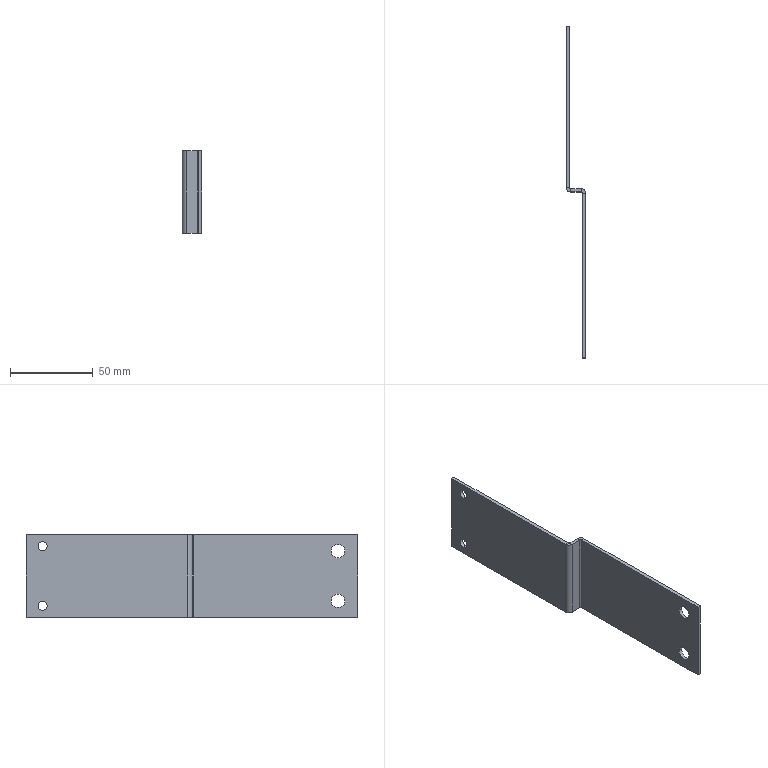Component | SolidWorks | JL001-05-01-010-2 | 1 solid | 30 faces | box 12 x 200 x 50 mm | volume 20545 mm3 | plane 18 | cylinder 12 | commonest cylinder face diameters 8.2 x4 5.5 x4 1.473 x2 5.473 x2
STEP:
#1=COLOUR_RGB('',0.7922,0.8196,0.9333);
#2=FILL_AREA_STYLE_COLOUR('',#1);
#3=FILL_AREA_STYLE('',(#2));
#4=SURFACE_STYLE_FILL_AREA(#3);
#5=SURFACE_SIDE_STYLE('',(#4));
#6=SURFACE_STYLE_USAGE(.BOTH.,#5);
#7=PRESENTATION_STYLE_ASSIGNMENT((#6));
#8=CARTESIAN_POINT('',(1.181,37.319,-0.4724));
#9=VERTEX_POINT('',#8);
#10=CARTESIAN_POINT('',(1.181,37.642,-0.4724));
#11=VERTEX_POINT('',#10);
#12=CARTESIAN_POINT('',(1.181,37.48,-0.4724));
#13=DIRECTION('',(-1.,0.,0.));
#14=DIRECTION('',(0.,1.,0.));
#15=AXIS2_PLACEMENT_3D('',#12,#13,#14);
#16=CIRCLE('',#15,0.1614);
#17=EDGE_CURVE('',#9,#11,#16,.T.);
#18=ORIENTED_EDGE('',*,*,#17,.T.);
#19=CARTESIAN_POINT('',(1.26,37.642,-0.4724));
#20=VERTEX_POINT('',#19);
#21=CARTESIAN_POINT('',(1.26,37.642,-0.4724));
#22=DIRECTION('',(1.,-0.,-0.));
#23=VECTOR('',#22,39.37);
#24=LINE('',#21,#23);
#25=EDGE_CURVE('',#11,#20,#24,.T.);
#26=ORIENTED_EDGE('',*,*,#25,.T.);
#27=CARTESIAN_POINT('',(1.26,37.319,-0.4724));
#28=VERTEX_POINT('',#27);
#29=CARTESIAN_POINT('',(1.26,37.48,-0.4724));
#30=DIRECTION('',(1.,-0.,-0.));
#31=DIRECTION('',(0.,-1.,0.));
#32=AXIS2_PLACEMENT_3D('',#29,#30,#31);
#33=CIRCLE('',#32,0.1614);
#34=EDGE_CURVE('',#20,#28,#33,.T.);
#35=ORIENTED_EDGE('',*,*,#34,.T.);
#36=CARTESIAN_POINT('',(1.26,37.319,-0.4724));
#37=DIRECTION('',(1.,-0.,-0.));
#38=VECTOR('',#37,39.37);
#39=LINE('',#36,#38);
#40=EDGE_CURVE('',#9,#28,#39,.T.);
#41=ORIENTED_EDGE('',*,*,#40,.F.);
#42=EDGE_LOOP('',(#18,#26,#35,#41));
#43=FACE_OUTER_BOUND('',#42,.T.);
#44=CARTESIAN_POINT('',(1.26,37.48,-0.4724));
#45=DIRECTION('',(1.,-0.,-0.));
#46=DIRECTION('',(0.,-1.,0.));
#47=AXIS2_PLACEMENT_3D('',#44,#45,#46);
#48=CYLINDRICAL_SURFACE('',#47,0.1614);
#49=ADVANCED_FACE('',(#43),#48,.F.);
#50=CARTESIAN_POINT('',(1.181,37.319,0.7087));
#51=VERTEX_POINT('',#50);
#52=CARTESIAN_POINT('',(1.181,37.642,0.7087));
#53=VERTEX_POINT('',#52);
#54=CARTESIAN_POINT('',(1.181,37.48,0.7087));
#55=DIRECTION('',(-1.,0.,0.));
#56=DIRECTION('',(0.,1.,0.));
#57=AXIS2_PLACEMENT_3D('',#54,#55,#56);
#58=CIRCLE('',#57,0.1614);
#59=EDGE_CURVE('',#51,#53,#58,.T.);
#60=ORIENTED_EDGE('',*,*,#59,.T.);
#61=CARTESIAN_POINT('',(1.26,37.642,0.7087));
#62=VERTEX_POINT('',#61);
#63=CARTESIAN_POINT('',(1.26,37.642,0.7087));
#64=DIRECTION('',(1.,-0.,-0.));
#65=VECTOR('',#64,39.37);
#66=LINE('',#63,#65);
#67=EDGE_CURVE('',#53,#62,#66,.T.);
#68=ORIENTED_EDGE('',*,*,#67,.T.);
#69=CARTESIAN_POINT('',(1.26,37.319,0.7087));
#70=VERTEX_POINT('',#69);
#71=CARTESIAN_POINT('',(1.26,37.48,0.7087));
#72=DIRECTION('',(1.,-0.,-0.));
#73=DIRECTION('',(0.,-1.,0.));
#74=AXIS2_PLACEMENT_3D('',#71,#72,#73);
#75=CIRCLE('',#74,0.1614);
#76=EDGE_CURVE('',#62,#70,#75,.T.);
#77=ORIENTED_EDGE('',*,*,#76,.T.);
#78=CARTESIAN_POINT('',(1.26,37.319,0.7087));
#79=DIRECTION('',(1.,-0.,-0.));
#80=VECTOR('',#79,39.37);
#81=LINE('',#78,#80);
#82=EDGE_CURVE('',#51,#70,#81,.T.);
#83=ORIENTED_EDGE('',*,*,#82,.F.);
#84=EDGE_LOOP('',(#60,#68,#77,#83));
#85=FACE_OUTER_BOUND('',#84,.T.);
#86=CARTESIAN_POINT('',(1.26,37.48,0.7087));
#87=DIRECTION('',(1.,-0.,-0.));
#88=DIRECTION('',(0.,-1.,0.));
#89=AXIS2_PLACEMENT_3D('',#86,#87,#88);
#90=CYLINDRICAL_SURFACE('',#89,0.1614);
#91=ADVANCED_FACE('',(#85),#90,.F.);
#92=CARTESIAN_POINT('',(0.7874,44.488,-0.6988));
#93=VERTEX_POINT('',#92);
#94=CARTESIAN_POINT('',(0.7874,44.488,-0.4823));
#95=VERTEX_POINT('',#94);
#96=CARTESIAN_POINT('',(0.7874,44.488,-0.5906));
#97=DIRECTION('',(1.,0.,-0.));
#98=DIRECTION('',(0.,0.,1.));
#99=AXIS2_PLACEMENT_3D('',#96,#97,#98);
#100=CIRCLE('',#99,0.1083);
#101=EDGE_CURVE('',#93,#95,#100,.T.);
#102=ORIENTED_EDGE('',*,*,#101,.F.);
#103=CARTESIAN_POINT('',(0.8661,44.488,-0.6988));
#104=VERTEX_POINT('',#103);
#105=CARTESIAN_POINT('',(0.8661,44.488,-0.6988));
#106=DIRECTION('',(1.,0.,-0.));
#107=VECTOR('',#106,39.37);
#108=LINE('',#105,#107);
#109=EDGE_CURVE('',#93,#104,#108,.T.);
#110=ORIENTED_EDGE('',*,*,#109,.T.);
#111=CARTESIAN_POINT('',(0.8661,44.488,-0.4823));
#112=VERTEX_POINT('',#111);
#113=CARTESIAN_POINT('',(0.8661,44.488,-0.5906));
#114=DIRECTION('',(1.,0.,-0.));
#115=DIRECTION('',(0.,0.,1.));
#116=AXIS2_PLACEMENT_3D('',#113,#114,#115);
#117=CIRCLE('',#116,0.1083);
#118=EDGE_CURVE('',#104,#112,#117,.T.);
#119=ORIENTED_EDGE('',*,*,#118,.T.);
#120=CARTESIAN_POINT('',(0.8661,44.488,-0.4823));
#121=DIRECTION('',(1.,0.,-0.));
#122=VECTOR('',#121,39.37);
#123=LINE('',#120,#122);
#124=EDGE_CURVE('',#95,#112,#123,.T.);
#125=ORIENTED_EDGE('',*,*,#124,.F.);
#126=EDGE_LOOP('',(#102,#110,#119,#125));
#127=FACE_OUTER_BOUND('',#126,.T.);
#128=CARTESIAN_POINT('',(0.8661,44.488,-0.5906));
#129=DIRECTION('',(1.,0.,-0.));
#130=DIRECTION('',(0.,0.,1.));
#131=AXIS2_PLACEMENT_3D('',#128,#129,#130);
#132=CYLINDRICAL_SURFACE('',#131,0.1083);
#133=ADVANCED_FACE('',(#127),#132,.F.);
#134=CARTESIAN_POINT('',(0.7874,44.488,0.7185));
#135=VERTEX_POINT('',#134);
#136=CARTESIAN_POINT('',(0.7874,44.488,0.935));
#137=VERTEX_POINT('',#136);
#138=CARTESIAN_POINT('',(0.7874,44.488,0.8268));
#139=DIRECTION('',(1.,0.,-0.));
#140=DIRECTION('',(0.,0.,1.));
#141=AXIS2_PLACEMENT_3D('',#138,#139,#140);
#142=CIRCLE('',#141,0.1083);
#143=EDGE_CURVE('',#135,#137,#142,.T.);
#144=ORIENTED_EDGE('',*,*,#143,.F.);
#145=CARTESIAN_POINT('',(0.8661,44.488,0.7185));
#146=VERTEX_POINT('',#145);
#147=CARTESIAN_POINT('',(0.8661,44.488,0.7185));
#148=DIRECTION('',(1.,0.,-0.));
#149=VECTOR('',#148,39.37);
#150=LINE('',#147,#149);
#151=EDGE_CURVE('',#135,#146,#150,.T.);
#152=ORIENTED_EDGE('',*,*,#151,.T.);
#153=CARTESIAN_POINT('',(0.8661,44.488,0.935));
#154=VERTEX_POINT('',#153);
#155=CARTESIAN_POINT('',(0.8661,44.488,0.8268));
#156=DIRECTION('',(1.,0.,-0.));
#157=DIRECTION('',(0.,0.,1.));
#158=AXIS2_PLACEMENT_3D('',#155,#156,#157);
#159=CIRCLE('',#158,0.1083);
#160=EDGE_CURVE('',#146,#154,#159,.T.);
#161=ORIENTED_EDGE('',*,*,#160,.T.);
#162=CARTESIAN_POINT('',(0.8661,44.488,0.935));
#163=DIRECTION('',(1.,0.,-0.));
#164=VECTOR('',#163,39.37);
#165=LINE('',#162,#164);
#166=EDGE_CURVE('',#137,#154,#165,.T.);
#167=ORIENTED_EDGE('',*,*,#166,.F.);
#168=EDGE_LOOP('',(#144,#152,#161,#167));
#169=FACE_OUTER_BOUND('',#168,.T.);
#170=CARTESIAN_POINT('',(0.8661,44.488,0.8268));
#171=DIRECTION('',(1.,0.,-0.));
#172=DIRECTION('',(0.,0.,1.));
#173=AXIS2_PLACEMENT_3D('',#170,#171,#172);
#174=CYLINDRICAL_SURFACE('',#173,0.1083);
#175=ADVANCED_FACE('',(#169),#174,.F.);
#176=CARTESIAN_POINT('',(0.8951,40.945,-0.8661));
#177=VERTEX_POINT('',#176);
#178=CARTESIAN_POINT('',(0.8951,41.024,-0.8661));
#179=VERTEX_POINT('',#178);
#180=CARTESIAN_POINT('',(0.8951,40.945,-0.8661));
#181=DIRECTION('',(0.,1.,0.));
#182=VECTOR('',#181,39.37);
#183=LINE('',#180,#182);
#184=EDGE_CURVE('',#177,#179,#183,.T.);
#185=ORIENTED_EDGE('',*,*,#184,.F.);
#186=CARTESIAN_POINT('',(0.7874,41.053,-0.8661));
#187=VERTEX_POINT('',#186);
#188=CARTESIAN_POINT('',(0.8951,41.053,-0.8661));
#189=DIRECTION('',(0.,0.,1.));
#190=DIRECTION('',(1.,0.,0.));
#191=AXIS2_PLACEMENT_3D('',#188,#189,#190);
#192=CIRCLE('',#191,0.1077);
#193=EDGE_CURVE('',#187,#177,#192,.T.);
#194=ORIENTED_EDGE('',*,*,#193,.F.);
#195=CARTESIAN_POINT('',(0.8661,41.053,-0.8661));
#196=VERTEX_POINT('',#195);
#197=CARTESIAN_POINT('',(0.8661,41.053,-0.8661));
#198=DIRECTION('',(-1.,0.,0.));
#199=VECTOR('',#198,39.37);
#200=LINE('',#197,#199);
#201=EDGE_CURVE('',#196,#187,#200,.T.);
#202=ORIENTED_EDGE('',*,*,#201,.F.);
#203=CARTESIAN_POINT('',(0.8951,41.053,-0.8661));
#204=DIRECTION('',(0.,0.,1.));
#205=DIRECTION('',(1.,0.,0.));
#206=AXIS2_PLACEMENT_3D('',#203,#204,#205);
#207=CIRCLE('',#206,0.029);
#208=EDGE_CURVE('',#196,#179,#207,.T.);
#209=ORIENTED_EDGE('',*,*,#208,.T.);
#210=EDGE_LOOP('',(#185,#194,#202,#209));
#211=FACE_OUTER_BOUND('',#210,.T.);
#212=CARTESIAN_POINT('',(0.8951,40.945,-0.8661));
#213=DIRECTION('',(-0.,0.,-1.));
#214=DIRECTION('',(1.,0.,-0.));
#215=AXIS2_PLACEMENT_3D('',#212,#213,#214);
#216=PLANE('',#215);
#217=ADVANCED_FACE('',(#211),#216,.T.);
#218=CARTESIAN_POINT('',(1.152,40.945,-0.8661));
#219=VERTEX_POINT('',#218);
#220=CARTESIAN_POINT('',(0.7874,40.945,-0.8661));
#221=DIRECTION('',(1.,0.,-0.));
#222=VECTOR('',#221,39.37);
#223=LINE('',#220,#222);
#224=EDGE_CURVE('',#177,#219,#223,.T.);
#225=ORIENTED_EDGE('',*,*,#224,.F.);
#226=ORIENTED_EDGE('',*,*,#184,.T.);
#227=CARTESIAN_POINT('',(1.152,41.024,-0.8661));
#228=VERTEX_POINT('',#227);
#229=CARTESIAN_POINT('',(0.7874,41.024,-0.8661));
#230=DIRECTION('',(1.,0.,-0.));
#231=VECTOR('',#230,39.37);
#232=LINE('',#229,#231);
#233=EDGE_CURVE('',#179,#228,#232,.T.);
#234=ORIENTED_EDGE('',*,*,#233,.T.);
#235=CARTESIAN_POINT('',(1.152,41.024,-0.8661));
#236=DIRECTION('',(0.,-1.,0.));
#237=VECTOR('',#236,39.37);
#238=LINE('',#235,#237);
#239=EDGE_CURVE('',#228,#219,#238,.T.);
#240=ORIENTED_EDGE('',*,*,#239,.T.);
#241=EDGE_LOOP('',(#225,#226,#234,#240));
#242=FACE_OUTER_BOUND('',#241,.T.);
#243=CARTESIAN_POINT('',(0.8661,41.053,-0.8661));
#244=DIRECTION('',(-0.,0.,-1.));
#245=DIRECTION('',(1.,0.,-0.));
#246=AXIS2_PLACEMENT_3D('',#243,#244,#245);
#247=PLANE('',#246);
#248=ADVANCED_FACE('',(#242),#247,.T.);
#249=CARTESIAN_POINT('',(0.7874,41.053,1.102));
#250=VERTEX_POINT('',#249);
#251=CARTESIAN_POINT('',(0.8661,41.053,1.102));
#252=VERTEX_POINT('',#251);
#253=CARTESIAN_POINT('',(0.7874,41.053,1.102));
#254=DIRECTION('',(1.,0.,-0.));
#255=VECTOR('',#254,39.37);
#256=LINE('',#253,#255);
#257=EDGE_CURVE('',#250,#252,#256,.T.);
#258=ORIENTED_EDGE('',*,*,#257,.F.);
#259=CARTESIAN_POINT('',(0.8951,40.945,1.102));
#260=VERTEX_POINT('',#259);
#261=CARTESIAN_POINT('',(0.8951,41.053,1.102));
#262=DIRECTION('',(0.,0.,1.));
#263=DIRECTION('',(1.,0.,0.));
#264=AXIS2_PLACEMENT_3D('',#261,#262,#263);
#265=CIRCLE('',#264,0.1077);
#266=EDGE_CURVE('',#250,#260,#265,.T.);
#267=ORIENTED_EDGE('',*,*,#266,.T.);
#268=CARTESIAN_POINT('',(0.8951,41.024,1.102));
#269=VERTEX_POINT('',#268);
#270=CARTESIAN_POINT('',(0.8951,41.024,1.102));
#271=DIRECTION('',(0.,-1.,0.));
#272=VECTOR('',#271,39.37);
#273=LINE('',#270,#272);
#274=EDGE_CURVE('',#269,#260,#273,.T.);
#275=ORIENTED_EDGE('',*,*,#274,.F.);
#276=CARTESIAN_POINT('',(0.8951,41.053,1.102));
#277=DIRECTION('',(0.,0.,1.));
#278=DIRECTION('',(1.,0.,0.));
#279=AXIS2_PLACEMENT_3D('',#276,#277,#278);
#280=CIRCLE('',#279,0.029);
#281=EDGE_CURVE('',#252,#269,#280,.T.);
#282=ORIENTED_EDGE('',*,*,#281,.F.);
#283=EDGE_LOOP('',(#258,#267,#275,#282));
#284=FACE_OUTER_BOUND('',#283,.T.);
#285=CARTESIAN_POINT('',(0.7874,41.053,1.102));
#286=DIRECTION('',(0.,0.,1.));
#287=DIRECTION('',(-1.,0.,0.));
#288=AXIS2_PLACEMENT_3D('',#285,#286,#287);
#289=PLANE('',#288);
#290=ADVANCED_FACE('',(#284),#289,.T.);
#291=CARTESIAN_POINT('',(0.7874,44.882,1.102));
#292=VERTEX_POINT('',#291);
#293=CARTESIAN_POINT('',(0.7874,44.882,1.102));
#294=DIRECTION('',(0.,-1.,0.));
#295=VECTOR('',#294,39.37);
#296=LINE('',#293,#295);
#297=EDGE_CURVE('',#292,#250,#296,.T.);
#298=ORIENTED_EDGE('',*,*,#297,.T.);
#299=ORIENTED_EDGE('',*,*,#257,.T.);
#300=CARTESIAN_POINT('',(0.8661,44.882,1.102));
#301=VERTEX_POINT('',#300);
#302=CARTESIAN_POINT('',(0.8661,44.882,1.102));
#303=DIRECTION('',(0.,-1.,0.));
#304=VECTOR('',#303,39.37);
#305=LINE('',#302,#304);
#306=EDGE_CURVE('',#301,#252,#305,.T.);
#307=ORIENTED_EDGE('',*,*,#306,.F.);
#308=CARTESIAN_POINT('',(0.8661,44.882,1.102));
#309=DIRECTION('',(-1.,0.,0.));
#310=VECTOR('',#309,39.37);
#311=LINE('',#308,#310);
#312=EDGE_CURVE('',#301,#292,#311,.T.);
#313=ORIENTED_EDGE('',*,*,#312,.T.);
#314=EDGE_LOOP('',(#298,#299,#307,#313));
#315=FACE_OUTER_BOUND('',#314,.T.);
#316=CARTESIAN_POINT('',(0.8951,41.024,1.102));
#317=DIRECTION('',(0.,0.,1.));
#318=DIRECTION('',(-1.,0.,0.));
#319=AXIS2_PLACEMENT_3D('',#316,#317,#318);
#320=PLANE('',#319);
#321=ADVANCED_FACE('',(#315),#320,.T.);
#322=CARTESIAN_POINT('',(1.181,40.916,-0.8661));
#323=VERTEX_POINT('',#322);
#324=CARTESIAN_POINT('',(1.26,40.916,-0.8661));
#325=VERTEX_POINT('',#324);
#326=CARTESIAN_POINT('',(1.181,40.916,-0.8661));
#327=DIRECTION('',(1.,0.,-0.));
#328=VECTOR('',#327,39.37);
#329=LINE('',#326,#328);
#330=EDGE_CURVE('',#323,#325,#329,.T.);
#331=ORIENTED_EDGE('',*,*,#330,.F.);
#332=CARTESIAN_POINT('',(1.152,40.916,-0.8661));
#333=DIRECTION('',(-0.,0.,-1.));
#334=DIRECTION('',(-1.,0.,0.));
#335=AXIS2_PLACEMENT_3D('',#332,#333,#334);
#336=CIRCLE('',#335,0.029);
#337=EDGE_CURVE('',#219,#323,#336,.T.);
#338=ORIENTED_EDGE('',*,*,#337,.F.);
#339=ORIENTED_EDGE('',*,*,#239,.F.);
#340=CARTESIAN_POINT('',(1.152,40.916,-0.8661));
#341=DIRECTION('',(-0.,0.,-1.));
#342=DIRECTION('',(1.,0.,0.));
#343=AXIS2_PLACEMENT_3D('',#340,#341,#342);
#344=CIRCLE('',#343,0.1077);
#345=EDGE_CURVE('',#228,#325,#344,.T.);
#346=ORIENTED_EDGE('',*,*,#345,.T.);
#347=EDGE_LOOP('',(#331,#338,#339,#346));
#348=FACE_OUTER_BOUND('',#347,.T.);
#349=CARTESIAN_POINT('',(1.181,40.916,-0.8661));
#350=DIRECTION('',(-0.,0.,-1.));
#351=DIRECTION('',(1.,0.,-0.));
#352=AXIS2_PLACEMENT_3D('',#349,#350,#351);
#353=PLANE('',#352);
#354=ADVANCED_FACE('',(#348),#353,.T.);
#355=CARTESIAN_POINT('',(1.181,37.008,-0.8661));
#356=VERTEX_POINT('',#355);
#357=CARTESIAN_POINT('',(1.181,40.945,-0.8661));
#358=DIRECTION('',(-0.,-1.,0.));
#359=VECTOR('',#358,39.37);
#360=LINE('',#357,#359);
#361=EDGE_CURVE('',#323,#356,#360,.T.);
#362=ORIENTED_EDGE('',*,*,#361,.F.);
#363=ORIENTED_EDGE('',*,*,#330,.T.);
#364=CARTESIAN_POINT('',(1.26,37.008,-0.8661));
#365=VERTEX_POINT('',#364);
#366=CARTESIAN_POINT('',(1.26,40.945,-0.8661));
#367=DIRECTION('',(-0.,-1.,0.));
#368=VECTOR('',#367,39.37);
#369=LINE('',#366,#368);
#370=EDGE_CURVE('',#325,#365,#369,.T.);
#371=ORIENTED_EDGE('',*,*,#370,.T.);
#372=CARTESIAN_POINT('',(1.181,37.008,-0.8661));
#373=DIRECTION('',(1.,0.,-0.));
#374=VECTOR('',#373,39.37);
#375=LINE('',#372,#374);
#376=EDGE_CURVE('',#356,#365,#375,.T.);
#377=ORIENTED_EDGE('',*,*,#376,.F.);
#378=EDGE_LOOP('',(#362,#363,#371,#377));
#379=FACE_OUTER_BOUND('',#378,.T.);
#380=CARTESIAN_POINT('',(1.152,41.024,-0.8661));
#381=DIRECTION('',(-0.,0.,-1.));
#382=DIRECTION('',(1.,0.,-0.));
#383=AXIS2_PLACEMENT_3D('',#380,#381,#382);
#384=PLANE('',#383);
#385=ADVANCED_FACE('',(#379),#384,.T.);
#386=CARTESIAN_POINT('',(1.152,40.945,1.102));
#387=VERTEX_POINT('',#386);
#388=CARTESIAN_POINT('',(1.152,41.024,1.102));
#389=VERTEX_POINT('',#388);
#390=CARTESIAN_POINT('',(1.152,40.945,1.102));
#391=DIRECTION('',(0.,1.,0.));
#392=VECTOR('',#391,39.37);
#393=LINE('',#390,#392);
#394=EDGE_CURVE('',#387,#389,#393,.T.);
#395=ORIENTED_EDGE('',*,*,#394,.F.);
#396=CARTESIAN_POINT('',(1.181,40.916,1.102));
#397=VERTEX_POINT('',#396);
#398=CARTESIAN_POINT('',(1.152,40.916,1.102));
#399=DIRECTION('',(-0.,0.,-1.));
#400=DIRECTION('',(-1.,0.,0.));
#401=AXIS2_PLACEMENT_3D('',#398,#399,#400);
#402=CIRCLE('',#401,0.029);
#403=EDGE_CURVE('',#387,#397,#402,.T.);
#404=ORIENTED_EDGE('',*,*,#403,.T.);
#405=CARTESIAN_POINT('',(1.26,40.916,1.102));
#406=VERTEX_POINT('',#405);
#407=CARTESIAN_POINT('',(1.26,40.916,1.102));
#408=DIRECTION('',(-1.,0.,0.));
#409=VECTOR('',#408,39.37);
#410=LINE('',#407,#409);
#411=EDGE_CURVE('',#406,#397,#410,.T.);
#412=ORIENTED_EDGE('',*,*,#411,.F.);
#413=CARTESIAN_POINT('',(1.152,40.916,1.102));
#414=DIRECTION('',(-0.,0.,-1.));
#415=DIRECTION('',(1.,0.,0.));
#416=AXIS2_PLACEMENT_3D('',#413,#414,#415);
#417=CIRCLE('',#416,0.1077);
#418=EDGE_CURVE('',#389,#406,#417,.T.);
#419=ORIENTED_EDGE('',*,*,#418,.F.);
#420=EDGE_LOOP('',(#395,#404,#412,#419));
#421=FACE_OUTER_BOUND('',#420,.T.);
#422=CARTESIAN_POINT('',(1.152,40.945,1.102));
#423=DIRECTION('',(0.,0.,1.));
#424=DIRECTION('',(-1.,0.,0.));
#425=AXIS2_PLACEMENT_3D('',#422,#423,#424);
#426=PLANE('',#425);
#427=ADVANCED_FACE('',(#421),#426,.T.);
#428=CARTESIAN_POINT('',(0.7874,40.945,1.102));
#429=DIRECTION('',(1.,0.,-0.));
#430=VECTOR('',#429,39.37);
#431=LINE('',#428,#430);
#432=EDGE_CURVE('',#260,#387,#431,.T.);
#433=ORIENTED_EDGE('',*,*,#432,.T.);
#434=ORIENTED_EDGE('',*,*,#394,.T.);
#435=CARTESIAN_POINT('',(0.7874,41.024,1.102));
#436=DIRECTION('',(1.,0.,-0.));
#437=VECTOR('',#436,39.37);
#438=LINE('',#435,#437);
#439=EDGE_CURVE('',#269,#389,#438,.T.);
#440=ORIENTED_EDGE('',*,*,#439,.F.);
#441=ORIENTED_EDGE('',*,*,#274,.T.);
#442=EDGE_LOOP('',(#433,#434,#440,#441));
#443=FACE_OUTER_BOUND('',#442,.T.);
#444=CARTESIAN_POINT('',(1.26,40.916,1.102));
#445=DIRECTION('',(0.,0.,1.));
#446=DIRECTION('',(-1.,0.,0.));
#447=AXIS2_PLACEMENT_3D('',#444,#445,#446);
#448=PLANE('',#447);
#449=ADVANCED_FACE('',(#443),#448,.T.);
#450=CARTESIAN_POINT('',(1.26,37.48,-0.4724));
#451=DIRECTION('',(1.,-0.,-0.));
#452=DIRECTION('',(0.,-1.,0.));
#453=AXIS2_PLACEMENT_3D('',#450,#451,#452);
#454=CIRCLE('',#453,0.1614);
#455=EDGE_CURVE('',#28,#20,#454,.T.);
#456=ORIENTED_EDGE('',*,*,#455,.F.);
#457=ORIENTED_EDGE('',*,*,#34,.F.);
#458=EDGE_LOOP('',(#456,#457));
#459=FACE_BOUND('',#458,.T.);
#460=CARTESIAN_POINT('',(1.26,37.48,0.7087));
#461=DIRECTION('',(1.,-0.,-0.));
#462=DIRECTION('',(0.,-1.,0.));
#463=AXIS2_PLACEMENT_3D('',#460,#461,#462);
#464=CIRCLE('',#463,0.1614);
#465=EDGE_CURVE('',#70,#62,#464,.T.);
#466=ORIENTED_EDGE('',*,*,#465,.F.);
#467=ORIENTED_EDGE('',*,*,#76,.F.);
#468=EDGE_LOOP('',(#466,#467));
#469=FACE_BOUND('',#468,.T.);
#470=CARTESIAN_POINT('',(1.26,37.008,1.102));
#471=VERTEX_POINT('',#470);
#472=CARTESIAN_POINT('',(1.26,40.945,1.102));
#473=DIRECTION('',(-0.,-1.,0.));
#474=VECTOR('',#473,39.37);
#475=LINE('',#472,#474);
#476=EDGE_CURVE('',#406,#471,#475,.T.);
#477=ORIENTED_EDGE('',*,*,#476,.T.);
#478=CARTESIAN_POINT('',(1.26,37.008,-0.8661));
#479=DIRECTION('',(0.,0.,1.));
#480=VECTOR('',#479,39.37);
#481=LINE('',#478,#480);
#482=EDGE_CURVE('',#365,#471,#481,.T.);
#483=ORIENTED_EDGE('',*,*,#482,.F.);
#484=ORIENTED_EDGE('',*,*,#370,.F.);
#485=CARTESIAN_POINT('',(1.26,40.916,-0.8661));
#486=DIRECTION('',(0.,0.,1.));
#487=VECTOR('',#486,39.37);
#488=LINE('',#485,#487);
#489=EDGE_CURVE('',#325,#406,#488,.T.);
#490=ORIENTED_EDGE('',*,*,#489,.T.);
#491=EDGE_LOOP('',(#477,#483,#484,#490));
#492=FACE_OUTER_BOUND('',#491,.T.);
#493=CARTESIAN_POINT('',(1.26,40.945,-0.8661));
#494=DIRECTION('',(-1.,0.,0.));
#495=DIRECTION('',(0.,1.,-0.));
#496=AXIS2_PLACEMENT_3D('',#493,#494,#495);
#497=PLANE('',#496);
#498=ADVANCED_FACE('',(#459,#469,#492),#497,.F.);
#499=CARTESIAN_POINT('',(1.181,37.008,1.102));
#500=VERTEX_POINT('',#499);
#501=CARTESIAN_POINT('',(1.181,37.008,1.102));
#502=DIRECTION('',(1.,0.,-0.));
#503=VECTOR('',#502,39.37);
#504=LINE('',#501,#503);
#505=EDGE_CURVE('',#500,#471,#504,.T.);
#506=ORIENTED_EDGE('',*,*,#505,.F.);
#507=CARTESIAN_POINT('',(1.181,37.008,-0.8661));
#508=DIRECTION('',(0.,0.,1.));
#509=VECTOR('',#508,39.37);
#510=LINE('',#507,#509);
#511=EDGE_CURVE('',#356,#500,#510,.T.);
#512=ORIENTED_EDGE('',*,*,#511,.F.);
#513=ORIENTED_EDGE('',*,*,#376,.T.);
#514=ORIENTED_EDGE('',*,*,#482,.T.);
#515=EDGE_LOOP('',(#506,#512,#513,#514));
#516=FACE_OUTER_BOUND('',#515,.T.);
#517=CARTESIAN_POINT('',(1.181,37.008,-0.8661));
#518=DIRECTION('',(0.,-1.,0.));
#519=DIRECTION('',(-1.,0.,0.));
#520=AXIS2_PLACEMENT_3D('',#517,#518,#519);
#521=PLANE('',#520);
#522=ADVANCED_FACE('',(#516),#521,.T.);
#523=ORIENTED_EDGE('',*,*,#17,.F.);
#524=CARTESIAN_POINT('',(1.181,37.48,-0.4724));
#525=DIRECTION('',(-1.,0.,0.));
#526=DIRECTION('',(0.,1.,0.));
#527=AXIS2_PLACEMENT_3D('',#524,#525,#526);
#528=CIRCLE('',#527,0.1614);
#529=EDGE_CURVE('',#11,#9,#528,.T.);
#530=ORIENTED_EDGE('',*,*,#529,.F.);
#531=EDGE_LOOP('',(#523,#530));
#532=FACE_BOUND('',#531,.T.);
#533=ORIENTED_EDGE('',*,*,#59,.F.);
#534=CARTESIAN_POINT('',(1.181,37.48,0.7087));
#535=DIRECTION('',(-1.,0.,0.));
#536=DIRECTION('',(0.,1.,0.));
#537=AXIS2_PLACEMENT_3D('',#534,#535,#536);
#538=CIRCLE('',#537,0.1614);
#539=EDGE_CURVE('',#53,#51,#538,.T.);
#540=ORIENTED_EDGE('',*,*,#539,.F.);
#541=EDGE_LOOP('',(#533,#540));
#542=FACE_BOUND('',#541,.T.);
#543=CARTESIAN_POINT('',(1.181,40.945,1.102));
#544=DIRECTION('',(-0.,-1.,0.));
#545=VECTOR('',#544,39.37);
#546=LINE('',#543,#545);
#547=EDGE_CURVE('',#397,#500,#546,.T.);
#548=ORIENTED_EDGE('',*,*,#547,.F.);
#549=CARTESIAN_POINT('',(1.181,40.916,-0.8661));
#550=DIRECTION('',(0.,0.,1.));
#551=VECTOR('',#550,39.37);
#552=LINE('',#549,#551);
#553=EDGE_CURVE('',#323,#397,#552,.T.);
#554=ORIENTED_EDGE('',*,*,#553,.F.);
#555=ORIENTED_EDGE('',*,*,#361,.T.);
#556=ORIENTED_EDGE('',*,*,#511,.T.);
#557=EDGE_LOOP('',(#548,#554,#555,#556));
#558=FACE_OUTER_BOUND('',#557,.T.);
#559=CARTESIAN_POINT('',(1.181,40.945,-0.8661));
#560=DIRECTION('',(-1.,0.,0.));
#561=DIRECTION('',(0.,1.,-0.));
#562=AXIS2_PLACEMENT_3D('',#559,#560,#561);
#563=PLANE('',#562);
#564=ADVANCED_FACE('',(#532,#542,#558),#563,.T.);
#565=ORIENTED_EDGE('',*,*,#403,.F.);
#566=CARTESIAN_POINT('',(1.152,40.945,-0.8661));
#567=DIRECTION('',(0.,0.,1.));
#568=VECTOR('',#567,39.37);
#569=LINE('',#566,#568);
#570=EDGE_CURVE('',#219,#387,#569,.T.);
#571=ORIENTED_EDGE('',*,*,#570,.F.);
#572=ORIENTED_EDGE('',*,*,#337,.T.);
#573=ORIENTED_EDGE('',*,*,#553,.T.);
#574=EDGE_LOOP('',(#565,#571,#572,#573));
#575=FACE_OUTER_BOUND('',#574,.T.);
#576=CARTESIAN_POINT('',(1.152,40.916,-0.8661));
#577=DIRECTION('',(0.,0.,1.));
#578=DIRECTION('',(-1.,0.,0.));
#579=AXIS2_PLACEMENT_3D('',#576,#577,#578);
#580=CYLINDRICAL_SURFACE('',#579,0.029);
#581=ADVANCED_FACE('',(#575),#580,.F.);
#582=ORIENTED_EDGE('',*,*,#432,.F.);
#583=CARTESIAN_POINT('',(0.8951,40.945,-0.8661));
#584=DIRECTION('',(0.,0.,1.));
#585=VECTOR('',#584,39.37);
#586=LINE('',#583,#585);
#587=EDGE_CURVE('',#177,#260,#586,.T.);
#588=ORIENTED_EDGE('',*,*,#587,.F.);
#589=ORIENTED_EDGE('',*,*,#224,.T.);
#590=ORIENTED_EDGE('',*,*,#570,.T.);
#591=EDGE_LOOP('',(#582,#588,#589,#590));
#592=FACE_OUTER_BOUND('',#591,.T.);
#593=CARTESIAN_POINT('',(0.7874,40.945,-0.8661));
#594=DIRECTION('',(0.,-1.,0.));
#595=DIRECTION('',(-1.,0.,0.));
#596=AXIS2_PLACEMENT_3D('',#593,#594,#595);
#597=PLANE('',#596);
#598=ADVANCED_FACE('',(#592),#597,.T.);
#599=ORIENTED_EDGE('',*,*,#266,.F.);
#600=CARTESIAN_POINT('',(0.7874,41.053,-0.8661));
#601=DIRECTION('',(0.,0.,1.));
#602=VECTOR('',#601,39.37);
#603=LINE('',#600,#602);
#604=EDGE_CURVE('',#187,#250,#603,.T.);
#605=ORIENTED_EDGE('',*,*,#604,.F.);
#606=ORIENTED_EDGE('',*,*,#193,.T.);
#607=ORIENTED_EDGE('',*,*,#587,.T.);
#608=EDGE_LOOP('',(#599,#605,#606,#607));
#609=FACE_OUTER_BOUND('',#608,.T.);
#610=CARTESIAN_POINT('',(0.8951,41.053,-0.8661));
#611=DIRECTION('',(0.,0.,1.));
#612=DIRECTION('',(-1.,0.,0.));
#613=AXIS2_PLACEMENT_3D('',#610,#611,#612);
#614=CYLINDRICAL_SURFACE('',#613,0.1077);
#615=ADVANCED_FACE('',(#609),#614,.T.);
#616=CARTESIAN_POINT('',(0.7874,44.488,-0.5906));
#617=DIRECTION('',(1.,0.,-0.));
#618=DIRECTION('',(0.,0.,1.));
#619=AXIS2_PLACEMENT_3D('',#616,#617,#618);
#620=CIRCLE('',#619,0.1083);
#621=EDGE_CURVE('',#95,#93,#620,.T.);
#622=ORIENTED_EDGE('',*,*,#621,.T.);
#623=ORIENTED_EDGE('',*,*,#101,.T.);
#624=EDGE_LOOP('',(#622,#623));
#625=FACE_BOUND('',#624,.T.);
#626=CARTESIAN_POINT('',(0.7874,44.488,0.8268));
#627=DIRECTION('',(1.,0.,-0.));
#628=DIRECTION('',(0.,0.,1.));
#629=AXIS2_PLACEMENT_3D('',#626,#627,#628);
#630=CIRCLE('',#629,0.1083);
#631=EDGE_CURVE('',#137,#135,#630,.T.);
#632=ORIENTED_EDGE('',*,*,#631,.T.);
#633=ORIENTED_EDGE('',*,*,#143,.T.);
#634=EDGE_LOOP('',(#632,#633));
#635=FACE_BOUND('',#634,.T.);
#636=ORIENTED_EDGE('',*,*,#297,.F.);
#637=CARTESIAN_POINT('',(0.7874,44.882,-0.8661));
#638=VERTEX_POINT('',#637);
#639=CARTESIAN_POINT('',(0.7874,44.882,-0.8661));
#640=DIRECTION('',(0.,0.,1.));
#641=VECTOR('',#640,39.37);
#642=LINE('',#639,#641);
#643=EDGE_CURVE('',#638,#292,#642,.T.);
#644=ORIENTED_EDGE('',*,*,#643,.F.);
#645=CARTESIAN_POINT('',(0.7874,44.882,-0.8661));
#646=DIRECTION('',(0.,-1.,0.));
#647=VECTOR('',#646,39.37);
#648=LINE('',#645,#647);
#649=EDGE_CURVE('',#638,#187,#648,.T.);
#650=ORIENTED_EDGE('',*,*,#649,.T.);
#651=ORIENTED_EDGE('',*,*,#604,.T.);
#652=EDGE_LOOP('',(#636,#644,#650,#651));
#653=FACE_OUTER_BOUND('',#652,.T.);
#654=CARTESIAN_POINT('',(0.7874,44.882,-0.8661));
#655=DIRECTION('',(-1.,0.,0.));
#656=DIRECTION('',(-0.,0.,-1.));
#657=AXIS2_PLACEMENT_3D('',#654,#655,#656);
#658=PLANE('',#657);
#659=ADVANCED_FACE('',(#625,#635,#653),#658,.T.);
#660=ORIENTED_EDGE('',*,*,#312,.F.);
#661=CARTESIAN_POINT('',(0.8661,44.882,-0.8661));
#662=VERTEX_POINT('',#661);
#663=CARTESIAN_POINT('',(0.8661,44.882,-0.8661));
#664=DIRECTION('',(0.,0.,1.));
#665=VECTOR('',#664,39.37);
#666=LINE('',#663,#665);
#667=EDGE_CURVE('',#662,#301,#666,.T.);
#668=ORIENTED_EDGE('',*,*,#667,.F.);
#669=CARTESIAN_POINT('',(0.8661,44.882,-0.8661));
#670=DIRECTION('',(-1.,0.,0.));
#671=VECTOR('',#670,39.37);
#672=LINE('',#669,#671);
#673=EDGE_CURVE('',#662,#638,#672,.T.);
#674=ORIENTED_EDGE('',*,*,#673,.T.);
#675=ORIENTED_EDGE('',*,*,#643,.T.);
#676=EDGE_LOOP('',(#660,#668,#674,#675));
#677=FACE_OUTER_BOUND('',#676,.T.);
#678=CARTESIAN_POINT('',(0.8661,44.882,-0.8661));
#679=DIRECTION('',(0.,1.,0.));
#680=DIRECTION('',(1.,0.,-0.));
#681=AXIS2_PLACEMENT_3D('',#678,#679,#680);
#682=PLANE('',#681);
#683=ADVANCED_FACE('',(#677),#682,.T.);
#684=CARTESIAN_POINT('',(0.8661,44.488,-0.5906));
#685=DIRECTION('',(1.,0.,-0.));
#686=DIRECTION('',(0.,0.,1.));
#687=AXIS2_PLACEMENT_3D('',#684,#685,#686);
#688=CIRCLE('',#687,0.1083);
#689=EDGE_CURVE('',#112,#104,#688,.T.);
#690=ORIENTED_EDGE('',*,*,#689,.F.);
#691=ORIENTED_EDGE('',*,*,#118,.F.);
#692=EDGE_LOOP('',(#690,#691));
#693=FACE_BOUND('',#692,.T.);
#694=CARTESIAN_POINT('',(0.8661,44.488,0.8268));
#695=DIRECTION('',(1.,0.,-0.));
#696=DIRECTION('',(0.,0.,1.));
#697=AXIS2_PLACEMENT_3D('',#694,#695,#696);
#698=CIRCLE('',#697,0.1083);
#699=EDGE_CURVE('',#154,#146,#698,.T.);
#700=ORIENTED_EDGE('',*,*,#699,.F.);
#701=ORIENTED_EDGE('',*,*,#160,.F.);
#702=EDGE_LOOP('',(#700,#701));
#703=FACE_BOUND('',#702,.T.);
#704=ORIENTED_EDGE('',*,*,#306,.T.);
#705=CARTESIAN_POINT('',(0.8661,41.053,-0.8661));
#706=DIRECTION('',(0.,0.,1.));
#707=VECTOR('',#706,39.37);
#708=LINE('',#705,#707);
#709=EDGE_CURVE('',#196,#252,#708,.T.);
#710=ORIENTED_EDGE('',*,*,#709,.F.);
#711=CARTESIAN_POINT('',(0.8661,44.882,-0.8661));
#712=DIRECTION('',(0.,-1.,0.));
#713=VECTOR('',#712,39.37);
#714=LINE('',#711,#713);
#715=EDGE_CURVE('',#662,#196,#714,.T.);
#716=ORIENTED_EDGE('',*,*,#715,.F.);
#717=ORIENTED_EDGE('',*,*,#667,.T.);
#718=EDGE_LOOP('',(#704,#710,#716,#717));
#719=FACE_OUTER_BOUND('',#718,.T.);
#720=CARTESIAN_POINT('',(0.8661,44.882,-0.8661));
#721=DIRECTION('',(-1.,0.,0.));
#722=DIRECTION('',(-0.,0.,-1.));
#723=AXIS2_PLACEMENT_3D('',#720,#721,#722);
#724=PLANE('',#723);
#725=ADVANCED_FACE('',(#693,#703,#719),#724,.F.);
#726=ORIENTED_EDGE('',*,*,#281,.T.);
#727=CARTESIAN_POINT('',(0.8951,41.024,-0.8661));
#728=DIRECTION('',(0.,0.,1.));
#729=VECTOR('',#728,39.37);
#730=LINE('',#727,#729);
#731=EDGE_CURVE('',#179,#269,#730,.T.);
#732=ORIENTED_EDGE('',*,*,#731,.F.);
#733=ORIENTED_EDGE('',*,*,#208,.F.);
#734=ORIENTED_EDGE('',*,*,#709,.T.);
#735=EDGE_LOOP('',(#726,#732,#733,#734));
#736=FACE_OUTER_BOUND('',#735,.T.);
#737=CARTESIAN_POINT('',(0.8951,41.053,-0.8661));
#738=DIRECTION('',(0.,0.,1.));
#739=DIRECTION('',(-1.,0.,0.));
#740=AXIS2_PLACEMENT_3D('',#737,#738,#739);
#741=CYLINDRICAL_SURFACE('',#740,0.029);
#742=ADVANCED_FACE('',(#736),#741,.F.);
#743=ORIENTED_EDGE('',*,*,#439,.T.);
#744=CARTESIAN_POINT('',(1.152,41.024,-0.8661));
#745=DIRECTION('',(0.,0.,1.));
#746=VECTOR('',#745,39.37);
#747=LINE('',#744,#746);
#748=EDGE_CURVE('',#228,#389,#747,.T.);
#749=ORIENTED_EDGE('',*,*,#748,.F.);
#750=ORIENTED_EDGE('',*,*,#233,.F.);
#751=ORIENTED_EDGE('',*,*,#731,.T.);
#752=EDGE_LOOP('',(#743,#749,#750,#751));
#753=FACE_OUTER_BOUND('',#752,.T.);
#754=CARTESIAN_POINT('',(0.7874,41.024,-0.8661));
#755=DIRECTION('',(0.,-1.,0.));
#756=DIRECTION('',(-1.,0.,0.));
#757=AXIS2_PLACEMENT_3D('',#754,#755,#756);
#758=PLANE('',#757);
#759=ADVANCED_FACE('',(#753),#758,.F.);
#760=ORIENTED_EDGE('',*,*,#418,.T.);
#761=ORIENTED_EDGE('',*,*,#489,.F.);
#762=ORIENTED_EDGE('',*,*,#345,.F.);
#763=ORIENTED_EDGE('',*,*,#748,.T.);
#764=EDGE_LOOP('',(#760,#761,#762,#763));
#765=FACE_OUTER_BOUND('',#764,.T.);
#766=CARTESIAN_POINT('',(1.152,40.916,-0.8661));
#767=DIRECTION('',(0.,0.,1.));
#768=DIRECTION('',(-1.,0.,0.));
#769=AXIS2_PLACEMENT_3D('',#766,#767,#768);
#770=CYLINDRICAL_SURFACE('',#769,0.1077);
#771=ADVANCED_FACE('',(#765),#770,.T.);
#772=ORIENTED_EDGE('',*,*,#715,.T.);
#773=ORIENTED_EDGE('',*,*,#201,.T.);
#774=ORIENTED_EDGE('',*,*,#649,.F.);
#775=ORIENTED_EDGE('',*,*,#673,.F.);
#776=EDGE_LOOP('',(#772,#773,#774,#775));
#777=FACE_OUTER_BOUND('',#776,.T.);
#778=CARTESIAN_POINT('',(1.152,40.916,-0.8661));
#779=DIRECTION('',(0.,0.,1.));
#780=DIRECTION('',(-1.,0.,0.));
#781=AXIS2_PLACEMENT_3D('',#778,#779,#780);
#782=PLANE('',#781);
#783=ADVANCED_FACE('',(#777),#782,.F.);
#784=ORIENTED_EDGE('',*,*,#476,.F.);
#785=ORIENTED_EDGE('',*,*,#411,.T.);
#786=ORIENTED_EDGE('',*,*,#547,.T.);
#787=ORIENTED_EDGE('',*,*,#505,.T.);
#788=EDGE_LOOP('',(#784,#785,#786,#787));
#789=FACE_OUTER_BOUND('',#788,.T.);
#790=CARTESIAN_POINT('',(1.152,40.916,1.102));
#791=DIRECTION('',(0.,0.,1.));
#792=DIRECTION('',(-1.,0.,0.));
#793=AXIS2_PLACEMENT_3D('',#790,#791,#792);
#794=PLANE('',#793);
#795=ADVANCED_FACE('',(#789),#794,.T.);
#796=ORIENTED_EDGE('',*,*,#151,.F.);
#797=ORIENTED_EDGE('',*,*,#631,.F.);
#798=ORIENTED_EDGE('',*,*,#166,.T.);
#799=ORIENTED_EDGE('',*,*,#699,.T.);
#800=EDGE_LOOP('',(#796,#797,#798,#799));
#801=FACE_OUTER_BOUND('',#800,.T.);
#802=CARTESIAN_POINT('',(0.8661,44.488,0.8268));
#803=DIRECTION('',(1.,0.,-0.));
#804=DIRECTION('',(0.,0.,1.));
#805=AXIS2_PLACEMENT_3D('',#802,#803,#804);
#806=CYLINDRICAL_SURFACE('',#805,0.1083);
#807=ADVANCED_FACE('',(#801),#806,.F.);
#808=ORIENTED_EDGE('',*,*,#109,.F.);
#809=ORIENTED_EDGE('',*,*,#621,.F.);
#810=ORIENTED_EDGE('',*,*,#124,.T.);
#811=ORIENTED_EDGE('',*,*,#689,.T.);
#812=EDGE_LOOP('',(#808,#809,#810,#811));
#813=FACE_OUTER_BOUND('',#812,.T.);
#814=CARTESIAN_POINT('',(0.8661,44.488,-0.5906));
#815=DIRECTION('',(1.,0.,-0.));
#816=DIRECTION('',(0.,0.,1.));
#817=AXIS2_PLACEMENT_3D('',#814,#815,#816);
#818=CYLINDRICAL_SURFACE('',#817,0.1083);
#819=ADVANCED_FACE('',(#813),#818,.F.);
#820=ORIENTED_EDGE('',*,*,#67,.F.);
#821=ORIENTED_EDGE('',*,*,#539,.T.);
#822=ORIENTED_EDGE('',*,*,#82,.T.);
#823=ORIENTED_EDGE('',*,*,#465,.T.);
#824=EDGE_LOOP('',(#820,#821,#822,#823));
#825=FACE_OUTER_BOUND('',#824,.T.);
#826=CARTESIAN_POINT('',(1.26,37.48,0.7087));
#827=DIRECTION('',(1.,-0.,-0.));
#828=DIRECTION('',(0.,-1.,0.));
#829=AXIS2_PLACEMENT_3D('',#826,#827,#828);
#830=CYLINDRICAL_SURFACE('',#829,0.1614);
#831=ADVANCED_FACE('',(#825),#830,.F.);
#832=ORIENTED_EDGE('',*,*,#25,.F.);
#833=ORIENTED_EDGE('',*,*,#529,.T.);
#834=ORIENTED_EDGE('',*,*,#40,.T.);
#835=ORIENTED_EDGE('',*,*,#455,.T.);
#836=EDGE_LOOP('',(#832,#833,#834,#835));
#837=FACE_OUTER_BOUND('',#836,.T.);
#838=CARTESIAN_POINT('',(1.26,37.48,-0.4724));
#839=DIRECTION('',(1.,-0.,-0.));
#840=DIRECTION('',(0.,-1.,0.));
#841=AXIS2_PLACEMENT_3D('',#838,#839,#840);
#842=CYLINDRICAL_SURFACE('',#841,0.1614);
#843=ADVANCED_FACE('',(#837),#842,.F.);
#844=CLOSED_SHELL('',(#49,#91,#133,#175,#217,#248,#290,#321,#354,#385,#427,#449,#498,#522,#564,#581,#598,#615,#659,#683,#725,#742,#759,#771,#783,#795,#807,#819,#831,#843));
#845=MANIFOLD_SOLID_BREP('',#844);
#846=STYLED_ITEM('',(#7),#845);
#847=PRESENTATION_LAYER_ASSIGNMENT('','',(#846));
#848=(LENGTH_UNIT()NAMED_UNIT(*)SI_UNIT($,.METRE.));
#849=LENGTH_MEASURE_WITH_UNIT(LENGTH_MEASURE(0.0254),#848);
#850=DIMENSIONAL_EXPONENTS(1.,0.,0.,0.,0.,0.,0.);
#851=(CONVERSION_BASED_UNIT('',#849)LENGTH_UNIT()NAMED_UNIT(#850));
#852=UNCERTAINTY_MEASURE_WITH_UNIT(LENGTH_MEASURE(0.00001),#851,'','');
#853=(NAMED_UNIT(*)PLANE_ANGLE_UNIT()SI_UNIT($,.RADIAN.));
#854=(NAMED_UNIT(*)SI_UNIT($,.STERADIAN.)SOLID_ANGLE_UNIT());
#855=(GEOMETRIC_REPRESENTATION_CONTEXT(3)GLOBAL_UNCERTAINTY_ASSIGNED_CONTEXT((#852))GLOBAL_UNIT_ASSIGNED_CONTEXT((#851,#853,#854))REPRESENTATION_CONTEXT('',''));
#856=MECHANICAL_DESIGN_GEOMETRIC_PRESENTATION_REPRESENTATION('',(#846),#855);
#857=CARTESIAN_POINT('',(0.,0.,0.));
#858=DIRECTION('',(0.,0.,1.));
#859=DIRECTION('',(1.,0.,0.));
#860=AXIS2_PLACEMENT_3D('',#857,#858,#859);
#861=(LENGTH_UNIT()NAMED_UNIT(*)SI_UNIT($,.METRE.));
#862=LENGTH_MEASURE_WITH_UNIT(LENGTH_MEASURE(0.0254),#861);
#863=DIMENSIONAL_EXPONENTS(1.,0.,0.,0.,0.,0.,0.);
#864=(CONVERSION_BASED_UNIT('',#862)LENGTH_UNIT()NAMED_UNIT(#863));
#865=UNCERTAINTY_MEASURE_WITH_UNIT(LENGTH_MEASURE(0.00001),#864,'','');
#866=(NAMED_UNIT(*)PLANE_ANGLE_UNIT()SI_UNIT($,.RADIAN.));
#867=(NAMED_UNIT(*)SI_UNIT($,.STERADIAN.)SOLID_ANGLE_UNIT());
#868=(GEOMETRIC_REPRESENTATION_CONTEXT(3)GLOBAL_UNCERTAINTY_ASSIGNED_CONTEXT((#865))GLOBAL_UNIT_ASSIGNED_CONTEXT((#864,#866,#867))REPRESENTATION_CONTEXT('',''));
#869=ADVANCED_BREP_SHAPE_REPRESENTATION('',(#845,#860),#868);